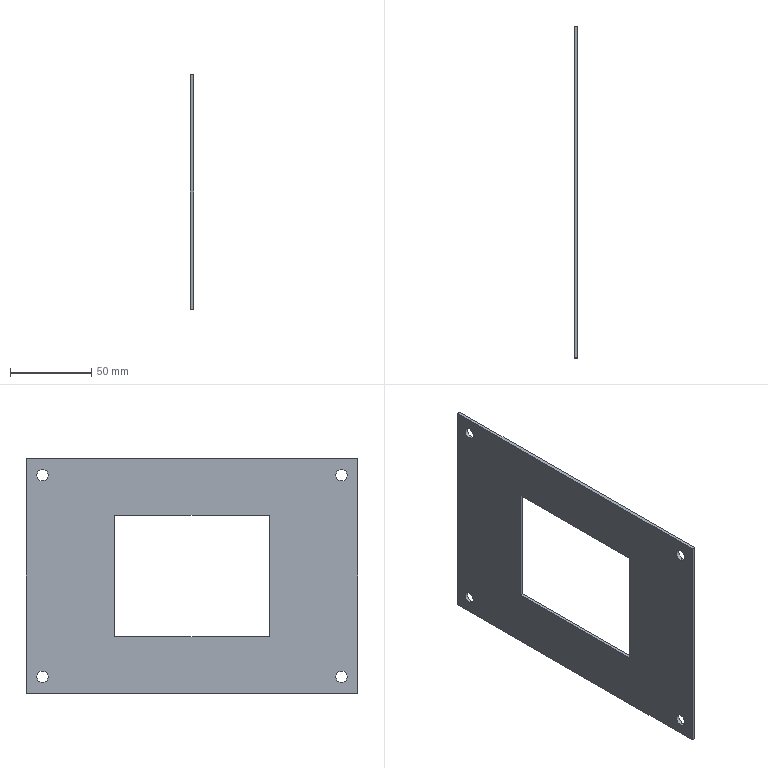Component | SolidWorks | TransformerBoxAssembly-1_TransformerBoxPlate-1 | 1 solid | 18 faces | box 2 x 204 x 144 mm | volume 44194 mm3 | plane 10 | cylinder 8 | commonest cylinder face diameters 7 x8
build123d program:
from build123d import *

# Parameters (mm, degrees)
SKETCH1_W           = 144
SKETCH1_H           = 204
SKETCH1_W_2         = 75
SKETCH1_H_2         = 95
BOSS_EXTRUDE1_DEPTH = 2
SKETCH2_R           = 3.5
CUT_EXTRUDE1_DEPTH  = 2


with BuildPart() as part:
    # Sketch1 → Boss-Extrude1 (new body)
    with BuildSketch(Plane.XY):
        with Locations((15.08, 2.278)):
            Rectangle(SKETCH1_W, SKETCH1_H)
        with Locations((15.08, 2.278)):
            Rectangle(SKETCH1_W_2, SKETCH1_H_2, mode=Mode.SUBTRACT)
    extrude(amount=BOSS_EXTRUDE1_DEPTH)

    # Sketch2 → Cut-Extrude1 (cut)
    with BuildSketch(Plane.XY.offset(2)):
        with Locations((-46.92, 94.278)):
            Circle(SKETCH2_R)
        with Locations((77.08, 94.278)):
            Circle(SKETCH2_R)
        with Locations((77.08, -89.722)):
            Circle(SKETCH2_R)
        with Locations((-46.92, -89.722)):
            Circle(SKETCH2_R)
    extrude(amount=-CUT_EXTRUDE1_DEPTH, mode=Mode.SUBTRACT)


solid = part.part

# Placed as in the assembly
solid = solid.moved(Location((-902.55, -140.711, -570.939), (0, 90, 0)))
STEP:
#1=CARTESIAN_POINT('',(-35.455,-9.072,-25.65));
#2=VERTEX_POINT('',#1);
#3=CARTESIAN_POINT('',(-35.455,-9.072,-25.375));
#4=VERTEX_POINT('',#3);
#5=CARTESIAN_POINT('',(-35.455,-9.072,-25.513));
#6=DIRECTION('',(-1.,0.,-0.));
#7=DIRECTION('',(0.,0.,1.));
#8=AXIS2_PLACEMENT_3D('',#5,#6,#7);
#9=CIRCLE('',#8,0.1378);
#10=EDGE_CURVE('',#2,#4,#9,.T.);
#11=ORIENTED_EDGE('',*,*,#10,.F.);
#12=CARTESIAN_POINT('',(-35.533,-9.072,-25.65));
#13=VERTEX_POINT('',#12);
#14=CARTESIAN_POINT('',(-35.455,-9.072,-25.65));
#15=DIRECTION('',(-1.,0.,-0.));
#16=VECTOR('',#15,39.37);
#17=LINE('',#14,#16);
#18=EDGE_CURVE('',#2,#13,#17,.T.);
#19=ORIENTED_EDGE('',*,*,#18,.T.);
#20=CARTESIAN_POINT('',(-35.533,-9.072,-25.375));
#21=VERTEX_POINT('',#20);
#22=CARTESIAN_POINT('',(-35.533,-9.072,-25.513));
#23=DIRECTION('',(-1.,0.,-0.));
#24=DIRECTION('',(0.,0.,1.));
#25=AXIS2_PLACEMENT_3D('',#22,#23,#24);
#26=CIRCLE('',#25,0.1378);
#27=EDGE_CURVE('',#13,#21,#26,.T.);
#28=ORIENTED_EDGE('',*,*,#27,.T.);
#29=CARTESIAN_POINT('',(-35.455,-9.072,-25.375));
#30=DIRECTION('',(-1.,0.,-0.));
#31=VECTOR('',#30,39.37);
#32=LINE('',#29,#31);
#33=EDGE_CURVE('',#4,#21,#32,.T.);
#34=ORIENTED_EDGE('',*,*,#33,.F.);
#35=EDGE_LOOP('',(#11,#19,#28,#34));
#36=FACE_OUTER_BOUND('',#35,.T.);
#37=CARTESIAN_POINT('',(-35.455,-9.072,-25.513));
#38=DIRECTION('',(-1.,0.,-0.));
#39=DIRECTION('',(0.,0.,1.));
#40=AXIS2_PLACEMENT_3D('',#37,#38,#39);
#41=CYLINDRICAL_SURFACE('',#40,0.1378);
#42=ADVANCED_FACE('',(#36),#41,.F.);
#43=CARTESIAN_POINT('',(-35.455,-9.072,-20.768));
#44=VERTEX_POINT('',#43);
#45=CARTESIAN_POINT('',(-35.455,-9.072,-20.493));
#46=VERTEX_POINT('',#45);
#47=CARTESIAN_POINT('',(-35.455,-9.072,-20.631));
#48=DIRECTION('',(-1.,0.,-0.));
#49=DIRECTION('',(0.,0.,1.));
#50=AXIS2_PLACEMENT_3D('',#47,#48,#49);
#51=CIRCLE('',#50,0.1378);
#52=EDGE_CURVE('',#44,#46,#51,.T.);
#53=ORIENTED_EDGE('',*,*,#52,.F.);
#54=CARTESIAN_POINT('',(-35.533,-9.072,-20.768));
#55=VERTEX_POINT('',#54);
#56=CARTESIAN_POINT('',(-35.455,-9.072,-20.768));
#57=DIRECTION('',(-1.,0.,-0.));
#58=VECTOR('',#57,39.37);
#59=LINE('',#56,#58);
#60=EDGE_CURVE('',#44,#55,#59,.T.);
#61=ORIENTED_EDGE('',*,*,#60,.T.);
#62=CARTESIAN_POINT('',(-35.533,-9.072,-20.493));
#63=VERTEX_POINT('',#62);
#64=CARTESIAN_POINT('',(-35.533,-9.072,-20.631));
#65=DIRECTION('',(-1.,0.,-0.));
#66=DIRECTION('',(0.,0.,1.));
#67=AXIS2_PLACEMENT_3D('',#64,#65,#66);
#68=CIRCLE('',#67,0.1378);
#69=EDGE_CURVE('',#55,#63,#68,.T.);
#70=ORIENTED_EDGE('',*,*,#69,.T.);
#71=CARTESIAN_POINT('',(-35.455,-9.072,-20.493));
#72=DIRECTION('',(-1.,0.,-0.));
#73=VECTOR('',#72,39.37);
#74=LINE('',#71,#73);
#75=EDGE_CURVE('',#46,#63,#74,.T.);
#76=ORIENTED_EDGE('',*,*,#75,.F.);
#77=EDGE_LOOP('',(#53,#61,#70,#76));
#78=FACE_OUTER_BOUND('',#77,.T.);
#79=CARTESIAN_POINT('',(-35.455,-9.072,-20.631));
#80=DIRECTION('',(-1.,0.,-0.));
#81=DIRECTION('',(0.,0.,1.));
#82=AXIS2_PLACEMENT_3D('',#79,#80,#81);
#83=CYLINDRICAL_SURFACE('',#82,0.1378);
#84=ADVANCED_FACE('',(#78),#83,.F.);
#85=CARTESIAN_POINT('',(-35.455,-1.828,-20.768));
#86=VERTEX_POINT('',#85);
#87=CARTESIAN_POINT('',(-35.455,-1.828,-20.493));
#88=VERTEX_POINT('',#87);
#89=CARTESIAN_POINT('',(-35.455,-1.828,-20.631));
#90=DIRECTION('',(-1.,0.,-0.));
#91=DIRECTION('',(0.,0.,1.));
#92=AXIS2_PLACEMENT_3D('',#89,#90,#91);
#93=CIRCLE('',#92,0.1378);
#94=EDGE_CURVE('',#86,#88,#93,.T.);
#95=ORIENTED_EDGE('',*,*,#94,.F.);
#96=CARTESIAN_POINT('',(-35.533,-1.828,-20.768));
#97=VERTEX_POINT('',#96);
#98=CARTESIAN_POINT('',(-35.455,-1.828,-20.768));
#99=DIRECTION('',(-1.,0.,-0.));
#100=VECTOR('',#99,39.37);
#101=LINE('',#98,#100);
#102=EDGE_CURVE('',#86,#97,#101,.T.);
#103=ORIENTED_EDGE('',*,*,#102,.T.);
#104=CARTESIAN_POINT('',(-35.533,-1.828,-20.493));
#105=VERTEX_POINT('',#104);
#106=CARTESIAN_POINT('',(-35.533,-1.828,-20.631));
#107=DIRECTION('',(-1.,0.,-0.));
#108=DIRECTION('',(0.,0.,1.));
#109=AXIS2_PLACEMENT_3D('',#106,#107,#108);
#110=CIRCLE('',#109,0.1378);
#111=EDGE_CURVE('',#97,#105,#110,.T.);
#112=ORIENTED_EDGE('',*,*,#111,.T.);
#113=CARTESIAN_POINT('',(-35.455,-1.828,-20.493));
#114=DIRECTION('',(-1.,0.,-0.));
#115=VECTOR('',#114,39.37);
#116=LINE('',#113,#115);
#117=EDGE_CURVE('',#88,#105,#116,.T.);
#118=ORIENTED_EDGE('',*,*,#117,.F.);
#119=EDGE_LOOP('',(#95,#103,#112,#118));
#120=FACE_OUTER_BOUND('',#119,.T.);
#121=CARTESIAN_POINT('',(-35.455,-1.828,-20.631));
#122=DIRECTION('',(-1.,0.,-0.));
#123=DIRECTION('',(0.,0.,1.));
#124=AXIS2_PLACEMENT_3D('',#121,#122,#123);
#125=CYLINDRICAL_SURFACE('',#124,0.1378);
#126=ADVANCED_FACE('',(#120),#125,.F.);
#127=CARTESIAN_POINT('',(-35.455,-1.828,-25.65));
#128=VERTEX_POINT('',#127);
#129=CARTESIAN_POINT('',(-35.455,-1.828,-25.375));
#130=VERTEX_POINT('',#129);
#131=CARTESIAN_POINT('',(-35.455,-1.828,-25.513));
#132=DIRECTION('',(-1.,0.,-0.));
#133=DIRECTION('',(0.,0.,1.));
#134=AXIS2_PLACEMENT_3D('',#131,#132,#133);
#135=CIRCLE('',#134,0.1378);
#136=EDGE_CURVE('',#128,#130,#135,.T.);
#137=ORIENTED_EDGE('',*,*,#136,.F.);
#138=CARTESIAN_POINT('',(-35.533,-1.828,-25.65));
#139=VERTEX_POINT('',#138);
#140=CARTESIAN_POINT('',(-35.455,-1.828,-25.65));
#141=DIRECTION('',(-1.,0.,-0.));
#142=VECTOR('',#141,39.37);
#143=LINE('',#140,#142);
#144=EDGE_CURVE('',#128,#139,#143,.T.);
#145=ORIENTED_EDGE('',*,*,#144,.T.);
#146=CARTESIAN_POINT('',(-35.533,-1.828,-25.375));
#147=VERTEX_POINT('',#146);
#148=CARTESIAN_POINT('',(-35.533,-1.828,-25.513));
#149=DIRECTION('',(-1.,0.,-0.));
#150=DIRECTION('',(0.,0.,1.));
#151=AXIS2_PLACEMENT_3D('',#148,#149,#150);
#152=CIRCLE('',#151,0.1378);
#153=EDGE_CURVE('',#139,#147,#152,.T.);
#154=ORIENTED_EDGE('',*,*,#153,.T.);
#155=CARTESIAN_POINT('',(-35.455,-1.828,-25.375));
#156=DIRECTION('',(-1.,0.,-0.));
#157=VECTOR('',#156,39.37);
#158=LINE('',#155,#157);
#159=EDGE_CURVE('',#130,#147,#158,.T.);
#160=ORIENTED_EDGE('',*,*,#159,.F.);
#161=EDGE_LOOP('',(#137,#145,#154,#160));
#162=FACE_OUTER_BOUND('',#161,.T.);
#163=CARTESIAN_POINT('',(-35.455,-1.828,-25.513));
#164=DIRECTION('',(-1.,0.,-0.));
#165=DIRECTION('',(0.,0.,1.));
#166=AXIS2_PLACEMENT_3D('',#163,#164,#165);
#167=CYLINDRICAL_SURFACE('',#166,0.1378);
#168=ADVANCED_FACE('',(#162),#167,.F.);
#169=CARTESIAN_POINT('',(-35.533,-9.072,-25.513));
#170=DIRECTION('',(-1.,0.,-0.));
#171=DIRECTION('',(0.,0.,1.));
#172=AXIS2_PLACEMENT_3D('',#169,#170,#171);
#173=CIRCLE('',#172,0.1378);
#174=EDGE_CURVE('',#21,#13,#173,.T.);
#175=ORIENTED_EDGE('',*,*,#174,.F.);
#176=ORIENTED_EDGE('',*,*,#27,.F.);
#177=EDGE_LOOP('',(#175,#176));
#178=FACE_BOUND('',#177,.T.);
#179=CARTESIAN_POINT('',(-35.533,-9.072,-20.631));
#180=DIRECTION('',(-1.,0.,-0.));
#181=DIRECTION('',(0.,0.,1.));
#182=AXIS2_PLACEMENT_3D('',#179,#180,#181);
#183=CIRCLE('',#182,0.1378);
#184=EDGE_CURVE('',#63,#55,#183,.T.);
#185=ORIENTED_EDGE('',*,*,#184,.F.);
#186=ORIENTED_EDGE('',*,*,#69,.F.);
#187=EDGE_LOOP('',(#185,#186));
#188=FACE_BOUND('',#187,.T.);
#189=CARTESIAN_POINT('',(-35.533,-1.828,-20.631));
#190=DIRECTION('',(-1.,0.,-0.));
#191=DIRECTION('',(0.,0.,1.));
#192=AXIS2_PLACEMENT_3D('',#189,#190,#191);
#193=CIRCLE('',#192,0.1378);
#194=EDGE_CURVE('',#105,#97,#193,.T.);
#195=ORIENTED_EDGE('',*,*,#194,.F.);
#196=ORIENTED_EDGE('',*,*,#111,.F.);
#197=EDGE_LOOP('',(#195,#196));
#198=FACE_BOUND('',#197,.T.);
#199=CARTESIAN_POINT('',(-35.533,-1.828,-25.513));
#200=DIRECTION('',(-1.,0.,-0.));
#201=DIRECTION('',(0.,0.,1.));
#202=AXIS2_PLACEMENT_3D('',#199,#200,#201);
#203=CIRCLE('',#202,0.1378);
#204=EDGE_CURVE('',#147,#139,#203,.T.);
#205=ORIENTED_EDGE('',*,*,#204,.F.);
#206=ORIENTED_EDGE('',*,*,#153,.F.);
#207=EDGE_LOOP('',(#205,#206));
#208=FACE_BOUND('',#207,.T.);
#209=CARTESIAN_POINT('',(-35.533,-1.434,-25.906));
#210=VERTEX_POINT('',#209);
#211=CARTESIAN_POINT('',(-35.533,-9.466,-25.906));
#212=VERTEX_POINT('',#211);
#213=CARTESIAN_POINT('',(-35.533,-1.434,-25.906));
#214=DIRECTION('',(-0.,-1.,-0.));
#215=VECTOR('',#214,39.37);
#216=LINE('',#213,#215);
#217=EDGE_CURVE('',#210,#212,#216,.T.);
#218=ORIENTED_EDGE('',*,*,#217,.T.);
#219=CARTESIAN_POINT('',(-35.533,-9.466,-20.237));
#220=VERTEX_POINT('',#219);
#221=CARTESIAN_POINT('',(-35.533,-9.466,-25.906));
#222=DIRECTION('',(0.,-0.,1.));
#223=VECTOR('',#222,39.37);
#224=LINE('',#221,#223);
#225=EDGE_CURVE('',#212,#220,#224,.T.);
#226=ORIENTED_EDGE('',*,*,#225,.T.);
#227=CARTESIAN_POINT('',(-35.533,-1.434,-20.237));
#228=VERTEX_POINT('',#227);
#229=CARTESIAN_POINT('',(-35.533,-1.434,-20.237));
#230=DIRECTION('',(0.,1.,0.));
#231=VECTOR('',#230,39.37);
#232=LINE('',#229,#231);
#233=EDGE_CURVE('',#220,#228,#232,.T.);
#234=ORIENTED_EDGE('',*,*,#233,.T.);
#235=CARTESIAN_POINT('',(-35.533,-1.434,-25.906));
#236=DIRECTION('',(-0.,0.,-1.));
#237=VECTOR('',#236,39.37);
#238=LINE('',#235,#237);
#239=EDGE_CURVE('',#228,#210,#238,.T.);
#240=ORIENTED_EDGE('',*,*,#239,.T.);
#241=EDGE_LOOP('',(#218,#226,#234,#240));
#242=FACE_OUTER_BOUND('',#241,.T.);
#243=CARTESIAN_POINT('',(-35.533,-7.32,-24.548));
#244=VERTEX_POINT('',#243);
#245=CARTESIAN_POINT('',(-35.533,-7.32,-21.595));
#246=VERTEX_POINT('',#245);
#247=CARTESIAN_POINT('',(-35.533,-7.32,-24.548));
#248=DIRECTION('',(0.,0.,1.));
#249=VECTOR('',#248,39.37);
#250=LINE('',#247,#249);
#251=EDGE_CURVE('',#244,#246,#250,.T.);
#252=ORIENTED_EDGE('',*,*,#251,.F.);
#253=CARTESIAN_POINT('',(-35.533,-3.58,-24.548));
#254=VERTEX_POINT('',#253);
#255=CARTESIAN_POINT('',(-35.533,-3.58,-24.548));
#256=DIRECTION('',(-0.,-1.,0.));
#257=VECTOR('',#256,39.37);
#258=LINE('',#255,#257);
#259=EDGE_CURVE('',#254,#244,#258,.T.);
#260=ORIENTED_EDGE('',*,*,#259,.F.);
#261=CARTESIAN_POINT('',(-35.533,-3.58,-21.595));
#262=VERTEX_POINT('',#261);
#263=CARTESIAN_POINT('',(-35.533,-3.58,-24.548));
#264=DIRECTION('',(-0.,0.,-1.));
#265=VECTOR('',#264,39.37);
#266=LINE('',#263,#265);
#267=EDGE_CURVE('',#262,#254,#266,.T.);
#268=ORIENTED_EDGE('',*,*,#267,.F.);
#269=CARTESIAN_POINT('',(-35.533,-3.58,-21.595));
#270=DIRECTION('',(0.,1.,-0.));
#271=VECTOR('',#270,39.37);
#272=LINE('',#269,#271);
#273=EDGE_CURVE('',#246,#262,#272,.T.);
#274=ORIENTED_EDGE('',*,*,#273,.F.);
#275=EDGE_LOOP('',(#252,#260,#268,#274));
#276=FACE_BOUND('',#275,.T.);
#277=CARTESIAN_POINT('',(-35.533,-5.54,-23.665));
#278=DIRECTION('',(-1.,0.,0.));
#279=DIRECTION('',(0.,-0.,1.));
#280=AXIS2_PLACEMENT_3D('',#277,#278,#279);
#281=PLANE('',#280);
#282=ADVANCED_FACE('',(#178,#188,#198,#208,#242,#276),#281,.T.);
#283=CARTESIAN_POINT('',(-35.455,-9.072,-25.513));
#284=DIRECTION('',(-1.,0.,-0.));
#285=DIRECTION('',(0.,0.,1.));
#286=AXIS2_PLACEMENT_3D('',#283,#284,#285);
#287=CIRCLE('',#286,0.1378);
#288=EDGE_CURVE('',#4,#2,#287,.T.);
#289=ORIENTED_EDGE('',*,*,#288,.T.);
#290=ORIENTED_EDGE('',*,*,#10,.T.);
#291=EDGE_LOOP('',(#289,#290));
#292=FACE_BOUND('',#291,.T.);
#293=CARTESIAN_POINT('',(-35.455,-9.072,-20.631));
#294=DIRECTION('',(-1.,0.,-0.));
#295=DIRECTION('',(0.,0.,1.));
#296=AXIS2_PLACEMENT_3D('',#293,#294,#295);
#297=CIRCLE('',#296,0.1378);
#298=EDGE_CURVE('',#46,#44,#297,.T.);
#299=ORIENTED_EDGE('',*,*,#298,.T.);
#300=ORIENTED_EDGE('',*,*,#52,.T.);
#301=EDGE_LOOP('',(#299,#300));
#302=FACE_BOUND('',#301,.T.);
#303=CARTESIAN_POINT('',(-35.455,-1.828,-20.631));
#304=DIRECTION('',(-1.,0.,-0.));
#305=DIRECTION('',(0.,0.,1.));
#306=AXIS2_PLACEMENT_3D('',#303,#304,#305);
#307=CIRCLE('',#306,0.1378);
#308=EDGE_CURVE('',#88,#86,#307,.T.);
#309=ORIENTED_EDGE('',*,*,#308,.T.);
#310=ORIENTED_EDGE('',*,*,#94,.T.);
#311=EDGE_LOOP('',(#309,#310));
#312=FACE_BOUND('',#311,.T.);
#313=CARTESIAN_POINT('',(-35.455,-1.828,-25.513));
#314=DIRECTION('',(-1.,0.,-0.));
#315=DIRECTION('',(0.,0.,1.));
#316=AXIS2_PLACEMENT_3D('',#313,#314,#315);
#317=CIRCLE('',#316,0.1378);
#318=EDGE_CURVE('',#130,#128,#317,.T.);
#319=ORIENTED_EDGE('',*,*,#318,.T.);
#320=ORIENTED_EDGE('',*,*,#136,.T.);
#321=EDGE_LOOP('',(#319,#320));
#322=FACE_BOUND('',#321,.T.);
#323=CARTESIAN_POINT('',(-35.455,-1.434,-25.906));
#324=VERTEX_POINT('',#323);
#325=CARTESIAN_POINT('',(-35.455,-9.466,-25.906));
#326=VERTEX_POINT('',#325);
#327=CARTESIAN_POINT('',(-35.455,-1.434,-25.906));
#328=DIRECTION('',(-0.,-1.,-0.));
#329=VECTOR('',#328,39.37);
#330=LINE('',#327,#329);
#331=EDGE_CURVE('',#324,#326,#330,.T.);
#332=ORIENTED_EDGE('',*,*,#331,.F.);
#333=CARTESIAN_POINT('',(-35.455,-1.434,-20.237));
#334=VERTEX_POINT('',#333);
#335=CARTESIAN_POINT('',(-35.455,-1.434,-25.906));
#336=DIRECTION('',(-0.,0.,-1.));
#337=VECTOR('',#336,39.37);
#338=LINE('',#335,#337);
#339=EDGE_CURVE('',#334,#324,#338,.T.);
#340=ORIENTED_EDGE('',*,*,#339,.F.);
#341=CARTESIAN_POINT('',(-35.455,-9.466,-20.237));
#342=VERTEX_POINT('',#341);
#343=CARTESIAN_POINT('',(-35.455,-1.434,-20.237));
#344=DIRECTION('',(0.,1.,0.));
#345=VECTOR('',#344,39.37);
#346=LINE('',#343,#345);
#347=EDGE_CURVE('',#342,#334,#346,.T.);
#348=ORIENTED_EDGE('',*,*,#347,.F.);
#349=CARTESIAN_POINT('',(-35.455,-9.466,-25.906));
#350=DIRECTION('',(0.,-0.,1.));
#351=VECTOR('',#350,39.37);
#352=LINE('',#349,#351);
#353=EDGE_CURVE('',#326,#342,#352,.T.);
#354=ORIENTED_EDGE('',*,*,#353,.F.);
#355=EDGE_LOOP('',(#332,#340,#348,#354));
#356=FACE_OUTER_BOUND('',#355,.T.);
#357=CARTESIAN_POINT('',(-35.455,-3.58,-24.548));
#358=VERTEX_POINT('',#357);
#359=CARTESIAN_POINT('',(-35.455,-7.32,-24.548));
#360=VERTEX_POINT('',#359);
#361=CARTESIAN_POINT('',(-35.455,-3.58,-24.548));
#362=DIRECTION('',(-0.,-1.,0.));
#363=VECTOR('',#362,39.37);
#364=LINE('',#361,#363);
#365=EDGE_CURVE('',#358,#360,#364,.T.);
#366=ORIENTED_EDGE('',*,*,#365,.T.);
#367=CARTESIAN_POINT('',(-35.455,-7.32,-21.595));
#368=VERTEX_POINT('',#367);
#369=CARTESIAN_POINT('',(-35.455,-7.32,-24.548));
#370=DIRECTION('',(0.,0.,1.));
#371=VECTOR('',#370,39.37);
#372=LINE('',#369,#371);
#373=EDGE_CURVE('',#360,#368,#372,.T.);
#374=ORIENTED_EDGE('',*,*,#373,.T.);
#375=CARTESIAN_POINT('',(-35.455,-3.58,-21.595));
#376=VERTEX_POINT('',#375);
#377=CARTESIAN_POINT('',(-35.455,-3.58,-21.595));
#378=DIRECTION('',(0.,1.,-0.));
#379=VECTOR('',#378,39.37);
#380=LINE('',#377,#379);
#381=EDGE_CURVE('',#368,#376,#380,.T.);
#382=ORIENTED_EDGE('',*,*,#381,.T.);
#383=CARTESIAN_POINT('',(-35.455,-3.58,-24.548));
#384=DIRECTION('',(-0.,0.,-1.));
#385=VECTOR('',#384,39.37);
#386=LINE('',#383,#385);
#387=EDGE_CURVE('',#376,#358,#386,.T.);
#388=ORIENTED_EDGE('',*,*,#387,.T.);
#389=EDGE_LOOP('',(#366,#374,#382,#388));
#390=FACE_BOUND('',#389,.T.);
#391=CARTESIAN_POINT('',(-35.455,-5.54,-23.665));
#392=DIRECTION('',(-1.,0.,0.));
#393=DIRECTION('',(0.,-0.,1.));
#394=AXIS2_PLACEMENT_3D('',#391,#392,#393);
#395=PLANE('',#394);
#396=ADVANCED_FACE('',(#292,#302,#312,#322,#356,#390),#395,.F.);
#397=ORIENTED_EDGE('',*,*,#331,.T.);
#398=CARTESIAN_POINT('',(-35.533,-9.466,-25.906));
#399=DIRECTION('',(1.,-0.,0.));
#400=VECTOR('',#399,39.37);
#401=LINE('',#398,#400);
#402=EDGE_CURVE('',#212,#326,#401,.T.);
#403=ORIENTED_EDGE('',*,*,#402,.F.);
#404=ORIENTED_EDGE('',*,*,#217,.F.);
#405=CARTESIAN_POINT('',(-35.533,-1.434,-25.906));
#406=DIRECTION('',(1.,-0.,0.));
#407=VECTOR('',#406,39.37);
#408=LINE('',#405,#407);
#409=EDGE_CURVE('',#210,#324,#408,.T.);
#410=ORIENTED_EDGE('',*,*,#409,.T.);
#411=EDGE_LOOP('',(#397,#403,#404,#410));
#412=FACE_OUTER_BOUND('',#411,.T.);
#413=CARTESIAN_POINT('',(-35.533,-1.434,-25.906));
#414=DIRECTION('',(0.,-0.,1.));
#415=DIRECTION('',(0.,1.,0.));
#416=AXIS2_PLACEMENT_3D('',#413,#414,#415);
#417=PLANE('',#416);
#418=ADVANCED_FACE('',(#412),#417,.F.);
#419=ORIENTED_EDGE('',*,*,#353,.T.);
#420=CARTESIAN_POINT('',(-35.533,-9.466,-20.237));
#421=DIRECTION('',(1.,-0.,0.));
#422=VECTOR('',#421,39.37);
#423=LINE('',#420,#422);
#424=EDGE_CURVE('',#220,#342,#423,.T.);
#425=ORIENTED_EDGE('',*,*,#424,.F.);
#426=ORIENTED_EDGE('',*,*,#225,.F.);
#427=ORIENTED_EDGE('',*,*,#402,.T.);
#428=EDGE_LOOP('',(#419,#425,#426,#427));
#429=FACE_OUTER_BOUND('',#428,.T.);
#430=CARTESIAN_POINT('',(-35.533,-9.466,-25.906));
#431=DIRECTION('',(0.,1.,0.));
#432=DIRECTION('',(-0.,0.,-1.));
#433=AXIS2_PLACEMENT_3D('',#430,#431,#432);
#434=PLANE('',#433);
#435=ADVANCED_FACE('',(#429),#434,.F.);
#436=ORIENTED_EDGE('',*,*,#347,.T.);
#437=CARTESIAN_POINT('',(-35.533,-1.434,-20.237));
#438=DIRECTION('',(1.,-0.,0.));
#439=VECTOR('',#438,39.37);
#440=LINE('',#437,#439);
#441=EDGE_CURVE('',#228,#334,#440,.T.);
#442=ORIENTED_EDGE('',*,*,#441,.F.);
#443=ORIENTED_EDGE('',*,*,#233,.F.);
#444=ORIENTED_EDGE('',*,*,#424,.T.);
#445=EDGE_LOOP('',(#436,#442,#443,#444));
#446=FACE_OUTER_BOUND('',#445,.T.);
#447=CARTESIAN_POINT('',(-35.533,-1.434,-20.237));
#448=DIRECTION('',(-0.,0.,-1.));
#449=DIRECTION('',(-0.,-1.,-0.));
#450=AXIS2_PLACEMENT_3D('',#447,#448,#449);
#451=PLANE('',#450);
#452=ADVANCED_FACE('',(#446),#451,.F.);
#453=ORIENTED_EDGE('',*,*,#339,.T.);
#454=ORIENTED_EDGE('',*,*,#409,.F.);
#455=ORIENTED_EDGE('',*,*,#239,.F.);
#456=ORIENTED_EDGE('',*,*,#441,.T.);
#457=EDGE_LOOP('',(#453,#454,#455,#456));
#458=FACE_OUTER_BOUND('',#457,.T.);
#459=CARTESIAN_POINT('',(-35.533,-1.434,-25.906));
#460=DIRECTION('',(-0.,-1.,-0.));
#461=DIRECTION('',(1.,-0.,0.));
#462=AXIS2_PLACEMENT_3D('',#459,#460,#461);
#463=PLANE('',#462);
#464=ADVANCED_FACE('',(#458),#463,.F.);
#465=ORIENTED_EDGE('',*,*,#365,.F.);
#466=CARTESIAN_POINT('',(-35.533,-3.58,-24.548));
#467=DIRECTION('',(1.,-0.,0.));
#468=VECTOR('',#467,39.37);
#469=LINE('',#466,#468);
#470=EDGE_CURVE('',#254,#358,#469,.T.);
#471=ORIENTED_EDGE('',*,*,#470,.F.);
#472=ORIENTED_EDGE('',*,*,#259,.T.);
#473=CARTESIAN_POINT('',(-35.533,-7.32,-24.548));
#474=DIRECTION('',(1.,-0.,0.));
#475=VECTOR('',#474,39.37);
#476=LINE('',#473,#475);
#477=EDGE_CURVE('',#244,#360,#476,.T.);
#478=ORIENTED_EDGE('',*,*,#477,.T.);
#479=EDGE_LOOP('',(#465,#471,#472,#478));
#480=FACE_OUTER_BOUND('',#479,.T.);
#481=CARTESIAN_POINT('',(-35.533,-3.58,-24.548));
#482=DIRECTION('',(0.,0.,1.));
#483=DIRECTION('',(0.,1.,-0.));
#484=AXIS2_PLACEMENT_3D('',#481,#482,#483);
#485=PLANE('',#484);
#486=ADVANCED_FACE('',(#480),#485,.T.);
#487=ORIENTED_EDGE('',*,*,#373,.F.);
#488=ORIENTED_EDGE('',*,*,#477,.F.);
#489=ORIENTED_EDGE('',*,*,#251,.T.);
#490=CARTESIAN_POINT('',(-35.533,-7.32,-21.595));
#491=DIRECTION('',(1.,-0.,0.));
#492=VECTOR('',#491,39.37);
#493=LINE('',#490,#492);
#494=EDGE_CURVE('',#246,#368,#493,.T.);
#495=ORIENTED_EDGE('',*,*,#494,.T.);
#496=EDGE_LOOP('',(#487,#488,#489,#495));
#497=FACE_OUTER_BOUND('',#496,.T.);
#498=CARTESIAN_POINT('',(-35.533,-7.32,-24.548));
#499=DIRECTION('',(0.,1.,-0.));
#500=DIRECTION('',(-0.,-0.,-1.));
#501=AXIS2_PLACEMENT_3D('',#498,#499,#500);
#502=PLANE('',#501);
#503=ADVANCED_FACE('',(#497),#502,.T.);
#504=ORIENTED_EDGE('',*,*,#381,.F.);
#505=ORIENTED_EDGE('',*,*,#494,.F.);
#506=ORIENTED_EDGE('',*,*,#273,.T.);
#507=CARTESIAN_POINT('',(-35.533,-3.58,-21.595));
#508=DIRECTION('',(1.,-0.,0.));
#509=VECTOR('',#508,39.37);
#510=LINE('',#507,#509);
#511=EDGE_CURVE('',#262,#376,#510,.T.);
#512=ORIENTED_EDGE('',*,*,#511,.T.);
#513=EDGE_LOOP('',(#504,#505,#506,#512));
#514=FACE_OUTER_BOUND('',#513,.T.);
#515=CARTESIAN_POINT('',(-35.533,-3.58,-21.595));
#516=DIRECTION('',(-0.,-0.,-1.));
#517=DIRECTION('',(-0.,-1.,0.));
#518=AXIS2_PLACEMENT_3D('',#515,#516,#517);
#519=PLANE('',#518);
#520=ADVANCED_FACE('',(#514),#519,.T.);
#521=ORIENTED_EDGE('',*,*,#387,.F.);
#522=ORIENTED_EDGE('',*,*,#511,.F.);
#523=ORIENTED_EDGE('',*,*,#267,.T.);
#524=ORIENTED_EDGE('',*,*,#470,.T.);
#525=EDGE_LOOP('',(#521,#522,#523,#524));
#526=FACE_OUTER_BOUND('',#525,.T.);
#527=CARTESIAN_POINT('',(-35.533,-3.58,-24.548));
#528=DIRECTION('',(-0.,-1.,-0.));
#529=DIRECTION('',(1.,-0.,0.));
#530=AXIS2_PLACEMENT_3D('',#527,#528,#529);
#531=PLANE('',#530);
#532=ADVANCED_FACE('',(#526),#531,.T.);
#533=ORIENTED_EDGE('',*,*,#144,.F.);
#534=ORIENTED_EDGE('',*,*,#318,.F.);
#535=ORIENTED_EDGE('',*,*,#159,.T.);
#536=ORIENTED_EDGE('',*,*,#204,.T.);
#537=EDGE_LOOP('',(#533,#534,#535,#536));
#538=FACE_OUTER_BOUND('',#537,.T.);
#539=CARTESIAN_POINT('',(-35.455,-1.828,-25.513));
#540=DIRECTION('',(-1.,0.,-0.));
#541=DIRECTION('',(0.,0.,1.));
#542=AXIS2_PLACEMENT_3D('',#539,#540,#541);
#543=CYLINDRICAL_SURFACE('',#542,0.1378);
#544=ADVANCED_FACE('',(#538),#543,.F.);
#545=ORIENTED_EDGE('',*,*,#102,.F.);
#546=ORIENTED_EDGE('',*,*,#308,.F.);
#547=ORIENTED_EDGE('',*,*,#117,.T.);
#548=ORIENTED_EDGE('',*,*,#194,.T.);
#549=EDGE_LOOP('',(#545,#546,#547,#548));
#550=FACE_OUTER_BOUND('',#549,.T.);
#551=CARTESIAN_POINT('',(-35.455,-1.828,-20.631));
#552=DIRECTION('',(-1.,0.,-0.));
#553=DIRECTION('',(0.,0.,1.));
#554=AXIS2_PLACEMENT_3D('',#551,#552,#553);
#555=CYLINDRICAL_SURFACE('',#554,0.1378);
#556=ADVANCED_FACE('',(#550),#555,.F.);
#557=ORIENTED_EDGE('',*,*,#60,.F.);
#558=ORIENTED_EDGE('',*,*,#298,.F.);
#559=ORIENTED_EDGE('',*,*,#75,.T.);
#560=ORIENTED_EDGE('',*,*,#184,.T.);
#561=EDGE_LOOP('',(#557,#558,#559,#560));
#562=FACE_OUTER_BOUND('',#561,.T.);
#563=CARTESIAN_POINT('',(-35.455,-9.072,-20.631));
#564=DIRECTION('',(-1.,0.,-0.));
#565=DIRECTION('',(0.,0.,1.));
#566=AXIS2_PLACEMENT_3D('',#563,#564,#565);
#567=CYLINDRICAL_SURFACE('',#566,0.1378);
#568=ADVANCED_FACE('',(#562),#567,.F.);
#569=ORIENTED_EDGE('',*,*,#18,.F.);
#570=ORIENTED_EDGE('',*,*,#288,.F.);
#571=ORIENTED_EDGE('',*,*,#33,.T.);
#572=ORIENTED_EDGE('',*,*,#174,.T.);
#573=EDGE_LOOP('',(#569,#570,#571,#572));
#574=FACE_OUTER_BOUND('',#573,.T.);
#575=CARTESIAN_POINT('',(-35.455,-9.072,-25.513));
#576=DIRECTION('',(-1.,0.,-0.));
#577=DIRECTION('',(0.,0.,1.));
#578=AXIS2_PLACEMENT_3D('',#575,#576,#577);
#579=CYLINDRICAL_SURFACE('',#578,0.1378);
#580=ADVANCED_FACE('',(#574),#579,.F.);
#581=CLOSED_SHELL('',(#42,#84,#126,#168,#282,#396,#418,#435,#452,#464,#486,#503,#520,#532,#544,#556,#568,#580));
#582=MANIFOLD_SOLID_BREP('',#581);
#583=CARTESIAN_POINT('',(0.,0.,0.));
#584=DIRECTION('',(0.,0.,1.));
#585=DIRECTION('',(1.,0.,0.));
#586=AXIS2_PLACEMENT_3D('',#583,#584,#585);
#587=(LENGTH_UNIT()NAMED_UNIT(*)SI_UNIT($,.METRE.));
#588=LENGTH_MEASURE_WITH_UNIT(LENGTH_MEASURE(0.0254),#587);
#589=DIMENSIONAL_EXPONENTS(1.,0.,0.,0.,0.,0.,0.);
#590=(CONVERSION_BASED_UNIT('',#588)LENGTH_UNIT()NAMED_UNIT(#589));
#591=UNCERTAINTY_MEASURE_WITH_UNIT(LENGTH_MEASURE(0.00001),#590,'','');
#592=(NAMED_UNIT(*)PLANE_ANGLE_UNIT()SI_UNIT($,.RADIAN.));
#593=(NAMED_UNIT(*)SI_UNIT($,.STERADIAN.)SOLID_ANGLE_UNIT());
#594=(GEOMETRIC_REPRESENTATION_CONTEXT(3)GLOBAL_UNCERTAINTY_ASSIGNED_CONTEXT((#591))GLOBAL_UNIT_ASSIGNED_CONTEXT((#590,#592,#593))REPRESENTATION_CONTEXT('',''));
#595=ADVANCED_BREP_SHAPE_REPRESENTATION('',(#582,#586),#594);
#596=COLOUR_RGB('',0.7922,0.8196,0.9333);
#597=FILL_AREA_STYLE_COLOUR('',#596);
#598=FILL_AREA_STYLE('',(#597));
#599=SURFACE_STYLE_FILL_AREA(#598);
#600=SURFACE_SIDE_STYLE('',(#599));
#601=SURFACE_STYLE_USAGE(.BOTH.,#600);
#602=PRESENTATION_STYLE_ASSIGNMENT((#601));
#603=STYLED_ITEM('',(#602),#582);
#604=PRESENTATION_LAYER_ASSIGNMENT('','',(#603));
#605=(LENGTH_UNIT()NAMED_UNIT(*)SI_UNIT($,.METRE.));
#606=LENGTH_MEASURE_WITH_UNIT(LENGTH_MEASURE(0.0254),#605);
#607=DIMENSIONAL_EXPONENTS(1.,0.,0.,0.,0.,0.,0.);
#608=(CONVERSION_BASED_UNIT('',#606)LENGTH_UNIT()NAMED_UNIT(#607));
#609=UNCERTAINTY_MEASURE_WITH_UNIT(LENGTH_MEASURE(0.00001),#608,'','');
#610=(NAMED_UNIT(*)PLANE_ANGLE_UNIT()SI_UNIT($,.RADIAN.));
#611=(NAMED_UNIT(*)SI_UNIT($,.STERADIAN.)SOLID_ANGLE_UNIT());
#612=(GEOMETRIC_REPRESENTATION_CONTEXT(3)GLOBAL_UNCERTAINTY_ASSIGNED_CONTEXT((#609))GLOBAL_UNIT_ASSIGNED_CONTEXT((#608,#610,#611))REPRESENTATION_CONTEXT('',''));
#613=MECHANICAL_DESIGN_GEOMETRIC_PRESENTATION_REPRESENTATION('',(#603),#612);